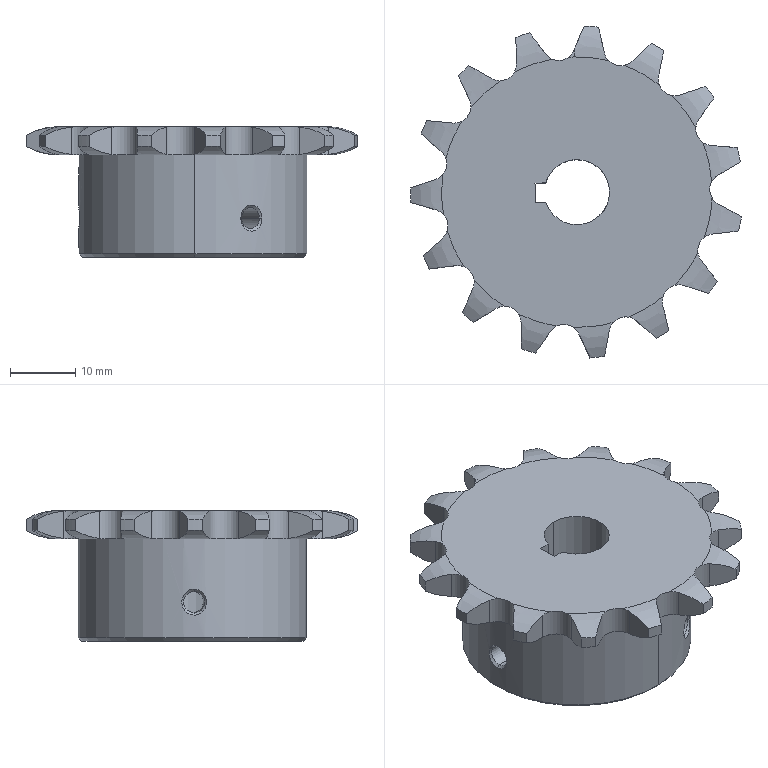Component | SolidWorks | LD101-02--Q1000-Q16-1.SLDQ1SM-1_LD101-02-35B15-d10-1 | 1 solid | 121 faces | volume 20009 mm3 | cylinder 44 | plane 39 | spline 32 | cone 6 | commonest cylinder face diameters 5.08 x20 51 x15 3.242 x4 10 x3 35 x2